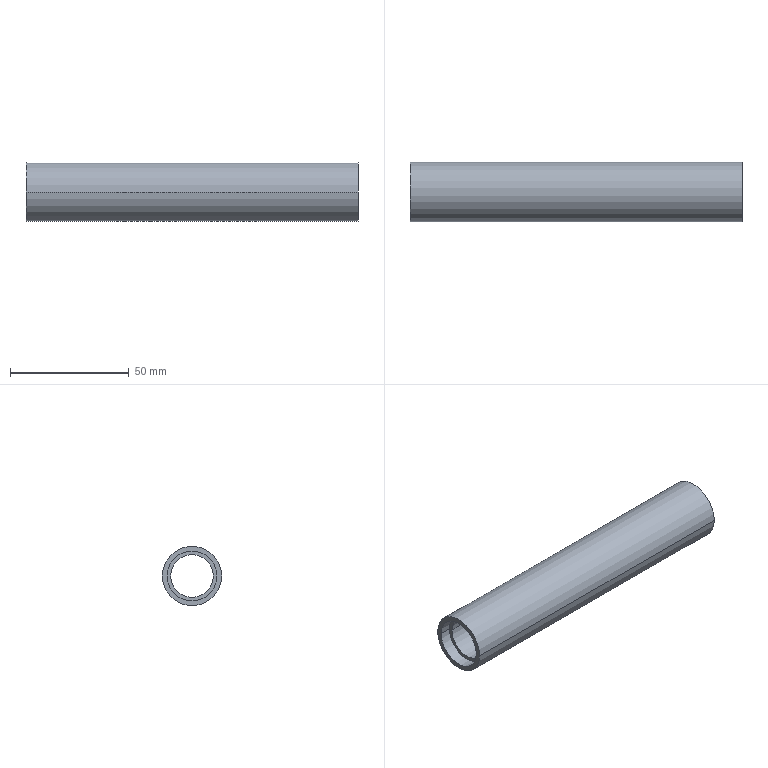Component | SolidWorks | IdlerAssembly4-1_Roller3-1 | 1 solid | 12 faces | box 140 x 25 x 25 mm | volume 32178 mm3 | cylinder 8 | plane 4 | commonest cylinder face diameters 21 x4 18 x2 25 x2
build123d program:
from build123d import *


with BuildPart() as part:
    # Sketch1 → Revolve1 (revolve)
    with BuildSketch(Plane.XY, mode=Mode.PRIVATE) as revolve1_sk:
        Polygon((0, 10.5), (5, 10.5), (5, 9), (135, 9), (135, 10.5), (140, 10.5), (140, 12.5), (0, 12.5), align=None)
    revolve(revolve1_sk.sketch.rotate(Axis((-1300.924, 0, 0), (1, 0, 0)), 90), axis=Axis((-1300.924, 0, 0), (1, 0, 0)))


solid = part.part

# Placed as in the assembly
solid = solid.moved(Location((-314.97, -95, 30), (0, 0, 0)))
STEP:
#1=CARTESIAN_POINT('',(-12.204,-3.327,1.181));
#2=VERTEX_POINT('',#1);
#3=CARTESIAN_POINT('',(-12.204,-4.154,1.181));
#4=VERTEX_POINT('',#3);
#5=CARTESIAN_POINT('',(-12.204,-3.74,1.181));
#6=DIRECTION('',(-1.,-0.,0.));
#7=DIRECTION('',(0.,-1.,0.));
#8=AXIS2_PLACEMENT_3D('',#5,#6,#7);
#9=CIRCLE('',#8,0.4134);
#10=EDGE_CURVE('',#2,#4,#9,.T.);
#11=ORIENTED_EDGE('',*,*,#10,.F.);
#12=CARTESIAN_POINT('',(-12.4,-3.327,1.181));
#13=VERTEX_POINT('',#12);
#14=CARTESIAN_POINT('',(-63.618,-3.327,1.181));
#15=DIRECTION('',(-1.,-0.,0.));
#16=VECTOR('',#15,39.37);
#17=LINE('',#14,#16);
#18=EDGE_CURVE('',#2,#13,#17,.T.);
#19=ORIENTED_EDGE('',*,*,#18,.T.);
#20=CARTESIAN_POINT('',(-12.4,-4.154,1.181));
#21=VERTEX_POINT('',#20);
#22=CARTESIAN_POINT('',(-12.4,-3.74,1.181));
#23=DIRECTION('',(-1.,-0.,0.));
#24=DIRECTION('',(0.,-1.,0.));
#25=AXIS2_PLACEMENT_3D('',#22,#23,#24);
#26=CIRCLE('',#25,0.4134);
#27=EDGE_CURVE('',#13,#21,#26,.T.);
#28=ORIENTED_EDGE('',*,*,#27,.T.);
#29=CARTESIAN_POINT('',(-63.618,-4.154,1.181));
#30=DIRECTION('',(-1.,-0.,0.));
#31=VECTOR('',#30,39.37);
#32=LINE('',#29,#31);
#33=EDGE_CURVE('',#4,#21,#32,.T.);
#34=ORIENTED_EDGE('',*,*,#33,.F.);
#35=EDGE_LOOP('',(#11,#19,#28,#34));
#36=FACE_OUTER_BOUND('',#35,.T.);
#37=CARTESIAN_POINT('',(-63.618,-3.74,1.181));
#38=DIRECTION('',(-1.,-0.,0.));
#39=DIRECTION('',(0.,-1.,0.));
#40=AXIS2_PLACEMENT_3D('',#37,#38,#39);
#41=CYLINDRICAL_SURFACE('',#40,0.4134);
#42=ADVANCED_FACE('',(#36),#41,.F.);
#43=CARTESIAN_POINT('',(-7.085,-3.386,1.181));
#44=VERTEX_POINT('',#43);
#45=CARTESIAN_POINT('',(-7.085,-4.094,1.181));
#46=VERTEX_POINT('',#45);
#47=CARTESIAN_POINT('',(-7.085,-3.74,1.181));
#48=DIRECTION('',(-1.,-0.,0.));
#49=DIRECTION('',(0.,-1.,0.));
#50=AXIS2_PLACEMENT_3D('',#47,#48,#49);
#51=CIRCLE('',#50,0.3543);
#52=EDGE_CURVE('',#44,#46,#51,.T.);
#53=ORIENTED_EDGE('',*,*,#52,.F.);
#54=CARTESIAN_POINT('',(-12.204,-3.386,1.181));
#55=VERTEX_POINT('',#54);
#56=CARTESIAN_POINT('',(-63.618,-3.386,1.181));
#57=DIRECTION('',(-1.,-0.,0.));
#58=VECTOR('',#57,39.37);
#59=LINE('',#56,#58);
#60=EDGE_CURVE('',#44,#55,#59,.T.);
#61=ORIENTED_EDGE('',*,*,#60,.T.);
#62=CARTESIAN_POINT('',(-12.204,-4.094,1.181));
#63=VERTEX_POINT('',#62);
#64=CARTESIAN_POINT('',(-12.204,-3.74,1.181));
#65=DIRECTION('',(-1.,-0.,0.));
#66=DIRECTION('',(0.,-1.,0.));
#67=AXIS2_PLACEMENT_3D('',#64,#65,#66);
#68=CIRCLE('',#67,0.3543);
#69=EDGE_CURVE('',#55,#63,#68,.T.);
#70=ORIENTED_EDGE('',*,*,#69,.T.);
#71=CARTESIAN_POINT('',(-63.618,-4.094,1.181));
#72=DIRECTION('',(-1.,-0.,0.));
#73=VECTOR('',#72,39.37);
#74=LINE('',#71,#73);
#75=EDGE_CURVE('',#46,#63,#74,.T.);
#76=ORIENTED_EDGE('',*,*,#75,.F.);
#77=EDGE_LOOP('',(#53,#61,#70,#76));
#78=FACE_OUTER_BOUND('',#77,.T.);
#79=CARTESIAN_POINT('',(-63.618,-3.74,1.181));
#80=DIRECTION('',(-1.,-0.,0.));
#81=DIRECTION('',(0.,-1.,0.));
#82=AXIS2_PLACEMENT_3D('',#79,#80,#81);
#83=CYLINDRICAL_SURFACE('',#82,0.3543);
#84=ADVANCED_FACE('',(#78),#83,.F.);
#85=CARTESIAN_POINT('',(-6.889,-3.327,1.181));
#86=VERTEX_POINT('',#85);
#87=CARTESIAN_POINT('',(-6.889,-4.154,1.181));
#88=VERTEX_POINT('',#87);
#89=CARTESIAN_POINT('',(-6.889,-3.74,1.181));
#90=DIRECTION('',(-1.,-0.,0.));
#91=DIRECTION('',(0.,-1.,0.));
#92=AXIS2_PLACEMENT_3D('',#89,#90,#91);
#93=CIRCLE('',#92,0.4134);
#94=EDGE_CURVE('',#86,#88,#93,.T.);
#95=ORIENTED_EDGE('',*,*,#94,.F.);
#96=CARTESIAN_POINT('',(-7.085,-3.327,1.181));
#97=VERTEX_POINT('',#96);
#98=CARTESIAN_POINT('',(-63.618,-3.327,1.181));
#99=DIRECTION('',(-1.,-0.,0.));
#100=VECTOR('',#99,39.37);
#101=LINE('',#98,#100);
#102=EDGE_CURVE('',#86,#97,#101,.T.);
#103=ORIENTED_EDGE('',*,*,#102,.T.);
#104=CARTESIAN_POINT('',(-7.085,-4.154,1.181));
#105=VERTEX_POINT('',#104);
#106=CARTESIAN_POINT('',(-7.085,-3.74,1.181));
#107=DIRECTION('',(-1.,-0.,0.));
#108=DIRECTION('',(0.,-1.,0.));
#109=AXIS2_PLACEMENT_3D('',#106,#107,#108);
#110=CIRCLE('',#109,0.4134);
#111=EDGE_CURVE('',#97,#105,#110,.T.);
#112=ORIENTED_EDGE('',*,*,#111,.T.);
#113=CARTESIAN_POINT('',(-63.618,-4.154,1.181));
#114=DIRECTION('',(-1.,-0.,0.));
#115=VECTOR('',#114,39.37);
#116=LINE('',#113,#115);
#117=EDGE_CURVE('',#88,#105,#116,.T.);
#118=ORIENTED_EDGE('',*,*,#117,.F.);
#119=EDGE_LOOP('',(#95,#103,#112,#118));
#120=FACE_OUTER_BOUND('',#119,.T.);
#121=CARTESIAN_POINT('',(-63.618,-3.74,1.181));
#122=DIRECTION('',(-1.,-0.,0.));
#123=DIRECTION('',(0.,-1.,0.));
#124=AXIS2_PLACEMENT_3D('',#121,#122,#123);
#125=CYLINDRICAL_SURFACE('',#124,0.4134);
#126=ADVANCED_FACE('',(#120),#125,.F.);
#127=CARTESIAN_POINT('',(-6.889,-4.232,1.181));
#128=VERTEX_POINT('',#127);
#129=CARTESIAN_POINT('',(-6.889,-3.248,1.181));
#130=VERTEX_POINT('',#129);
#131=CARTESIAN_POINT('',(-6.889,-3.74,1.181));
#132=DIRECTION('',(-1.,-0.,0.));
#133=DIRECTION('',(0.,-1.,0.));
#134=AXIS2_PLACEMENT_3D('',#131,#132,#133);
#135=CIRCLE('',#134,0.4921);
#136=EDGE_CURVE('',#128,#130,#135,.T.);
#137=ORIENTED_EDGE('',*,*,#136,.T.);
#138=CARTESIAN_POINT('',(-12.4,-3.248,1.181));
#139=VERTEX_POINT('',#138);
#140=CARTESIAN_POINT('',(-63.618,-3.248,1.181));
#141=DIRECTION('',(-1.,-0.,0.));
#142=VECTOR('',#141,39.37);
#143=LINE('',#140,#142);
#144=EDGE_CURVE('',#130,#139,#143,.T.);
#145=ORIENTED_EDGE('',*,*,#144,.T.);
#146=CARTESIAN_POINT('',(-12.4,-4.232,1.181));
#147=VERTEX_POINT('',#146);
#148=CARTESIAN_POINT('',(-12.4,-3.74,1.181));
#149=DIRECTION('',(-1.,-0.,0.));
#150=DIRECTION('',(0.,-1.,0.));
#151=AXIS2_PLACEMENT_3D('',#148,#149,#150);
#152=CIRCLE('',#151,0.4921);
#153=EDGE_CURVE('',#147,#139,#152,.T.);
#154=ORIENTED_EDGE('',*,*,#153,.F.);
#155=CARTESIAN_POINT('',(-63.618,-4.232,1.181));
#156=DIRECTION('',(-1.,-0.,0.));
#157=VECTOR('',#156,39.37);
#158=LINE('',#155,#157);
#159=EDGE_CURVE('',#128,#147,#158,.T.);
#160=ORIENTED_EDGE('',*,*,#159,.F.);
#161=EDGE_LOOP('',(#137,#145,#154,#160));
#162=FACE_OUTER_BOUND('',#161,.T.);
#163=CARTESIAN_POINT('',(-63.618,-3.74,1.181));
#164=DIRECTION('',(-1.,-0.,0.));
#165=DIRECTION('',(0.,-1.,0.));
#166=AXIS2_PLACEMENT_3D('',#163,#164,#165);
#167=CYLINDRICAL_SURFACE('',#166,0.4921);
#168=ADVANCED_FACE('',(#162),#167,.T.);
#169=CARTESIAN_POINT('',(-12.4,-3.74,1.181));
#170=DIRECTION('',(-1.,-0.,0.));
#171=DIRECTION('',(0.,-1.,0.));
#172=AXIS2_PLACEMENT_3D('',#169,#170,#171);
#173=CIRCLE('',#172,0.4134);
#174=EDGE_CURVE('',#21,#13,#173,.T.);
#175=ORIENTED_EDGE('',*,*,#174,.F.);
#176=ORIENTED_EDGE('',*,*,#27,.F.);
#177=EDGE_LOOP('',(#175,#176));
#178=FACE_BOUND('',#177,.T.);
#179=ORIENTED_EDGE('',*,*,#153,.T.);
#180=CARTESIAN_POINT('',(-12.4,-3.74,1.181));
#181=DIRECTION('',(-1.,-0.,0.));
#182=DIRECTION('',(0.,-1.,0.));
#183=AXIS2_PLACEMENT_3D('',#180,#181,#182);
#184=CIRCLE('',#183,0.4921);
#185=EDGE_CURVE('',#139,#147,#184,.T.);
#186=ORIENTED_EDGE('',*,*,#185,.T.);
#187=EDGE_LOOP('',(#179,#186));
#188=FACE_OUTER_BOUND('',#187,.T.);
#189=CARTESIAN_POINT('',(-12.4,-3.74,1.594));
#190=DIRECTION('',(1.,0.,-0.));
#191=DIRECTION('',(-0.,1.,0.));
#192=AXIS2_PLACEMENT_3D('',#189,#190,#191);
#193=PLANE('',#192);
#194=ADVANCED_FACE('',(#178,#188),#193,.F.);
#195=ORIENTED_EDGE('',*,*,#144,.F.);
#196=CARTESIAN_POINT('',(-6.889,-3.74,1.181));
#197=DIRECTION('',(-1.,-0.,0.));
#198=DIRECTION('',(0.,-1.,0.));
#199=AXIS2_PLACEMENT_3D('',#196,#197,#198);
#200=CIRCLE('',#199,0.4921);
#201=EDGE_CURVE('',#130,#128,#200,.T.);
#202=ORIENTED_EDGE('',*,*,#201,.T.);
#203=ORIENTED_EDGE('',*,*,#159,.T.);
#204=ORIENTED_EDGE('',*,*,#185,.F.);
#205=EDGE_LOOP('',(#195,#202,#203,#204));
#206=FACE_OUTER_BOUND('',#205,.T.);
#207=CARTESIAN_POINT('',(-63.618,-3.74,1.181));
#208=DIRECTION('',(-1.,-0.,0.));
#209=DIRECTION('',(0.,-1.,0.));
#210=AXIS2_PLACEMENT_3D('',#207,#208,#209);
#211=CYLINDRICAL_SURFACE('',#210,0.4921);
#212=ADVANCED_FACE('',(#206),#211,.T.);
#213=ORIENTED_EDGE('',*,*,#136,.F.);
#214=ORIENTED_EDGE('',*,*,#201,.F.);
#215=EDGE_LOOP('',(#213,#214));
#216=FACE_OUTER_BOUND('',#215,.T.);
#217=CARTESIAN_POINT('',(-6.889,-3.74,1.181));
#218=DIRECTION('',(-1.,-0.,0.));
#219=DIRECTION('',(0.,-1.,0.));
#220=AXIS2_PLACEMENT_3D('',#217,#218,#219);
#221=CIRCLE('',#220,0.4134);
#222=EDGE_CURVE('',#88,#86,#221,.T.);
#223=ORIENTED_EDGE('',*,*,#222,.T.);
#224=ORIENTED_EDGE('',*,*,#94,.T.);
#225=EDGE_LOOP('',(#223,#224));
#226=FACE_BOUND('',#225,.T.);
#227=CARTESIAN_POINT('',(-6.889,-3.74,1.673));
#228=DIRECTION('',(-1.,-0.,0.));
#229=DIRECTION('',(0.,-1.,0.));
#230=AXIS2_PLACEMENT_3D('',#227,#228,#229);
#231=PLANE('',#230);
#232=ADVANCED_FACE('',(#216,#226),#231,.F.);
#233=ORIENTED_EDGE('',*,*,#102,.F.);
#234=ORIENTED_EDGE('',*,*,#222,.F.);
#235=ORIENTED_EDGE('',*,*,#117,.T.);
#236=CARTESIAN_POINT('',(-7.085,-3.74,1.181));
#237=DIRECTION('',(-1.,-0.,0.));
#238=DIRECTION('',(0.,-1.,0.));
#239=AXIS2_PLACEMENT_3D('',#236,#237,#238);
#240=CIRCLE('',#239,0.4134);
#241=EDGE_CURVE('',#105,#97,#240,.T.);
#242=ORIENTED_EDGE('',*,*,#241,.T.);
#243=EDGE_LOOP('',(#233,#234,#235,#242));
#244=FACE_OUTER_BOUND('',#243,.T.);
#245=CARTESIAN_POINT('',(-63.618,-3.74,1.181));
#246=DIRECTION('',(-1.,-0.,0.));
#247=DIRECTION('',(0.,-1.,0.));
#248=AXIS2_PLACEMENT_3D('',#245,#246,#247);
#249=CYLINDRICAL_SURFACE('',#248,0.4134);
#250=ADVANCED_FACE('',(#244),#249,.F.);
#251=ORIENTED_EDGE('',*,*,#241,.F.);
#252=ORIENTED_EDGE('',*,*,#111,.F.);
#253=EDGE_LOOP('',(#251,#252));
#254=FACE_OUTER_BOUND('',#253,.T.);
#255=CARTESIAN_POINT('',(-7.085,-3.74,1.181));
#256=DIRECTION('',(-1.,-0.,0.));
#257=DIRECTION('',(0.,-1.,0.));
#258=AXIS2_PLACEMENT_3D('',#255,#256,#257);
#259=CIRCLE('',#258,0.3543);
#260=EDGE_CURVE('',#46,#44,#259,.T.);
#261=ORIENTED_EDGE('',*,*,#260,.T.);
#262=ORIENTED_EDGE('',*,*,#52,.T.);
#263=EDGE_LOOP('',(#261,#262));
#264=FACE_BOUND('',#263,.T.);
#265=CARTESIAN_POINT('',(-7.085,-3.74,1.535));
#266=DIRECTION('',(-1.,-0.,0.));
#267=DIRECTION('',(0.,-1.,0.));
#268=AXIS2_PLACEMENT_3D('',#265,#266,#267);
#269=PLANE('',#268);
#270=ADVANCED_FACE('',(#254,#264),#269,.F.);
#271=ORIENTED_EDGE('',*,*,#60,.F.);
#272=ORIENTED_EDGE('',*,*,#260,.F.);
#273=ORIENTED_EDGE('',*,*,#75,.T.);
#274=CARTESIAN_POINT('',(-12.204,-3.74,1.181));
#275=DIRECTION('',(-1.,-0.,0.));
#276=DIRECTION('',(0.,-1.,0.));
#277=AXIS2_PLACEMENT_3D('',#274,#275,#276);
#278=CIRCLE('',#277,0.3543);
#279=EDGE_CURVE('',#63,#55,#278,.T.);
#280=ORIENTED_EDGE('',*,*,#279,.T.);
#281=EDGE_LOOP('',(#271,#272,#273,#280));
#282=FACE_OUTER_BOUND('',#281,.T.);
#283=CARTESIAN_POINT('',(-63.618,-3.74,1.181));
#284=DIRECTION('',(-1.,-0.,0.));
#285=DIRECTION('',(0.,-1.,0.));
#286=AXIS2_PLACEMENT_3D('',#283,#284,#285);
#287=CYLINDRICAL_SURFACE('',#286,0.3543);
#288=ADVANCED_FACE('',(#282),#287,.F.);
#289=ORIENTED_EDGE('',*,*,#279,.F.);
#290=ORIENTED_EDGE('',*,*,#69,.F.);
#291=EDGE_LOOP('',(#289,#290));
#292=FACE_BOUND('',#291,.T.);
#293=CARTESIAN_POINT('',(-12.204,-3.74,1.181));
#294=DIRECTION('',(-1.,-0.,0.));
#295=DIRECTION('',(0.,-1.,0.));
#296=AXIS2_PLACEMENT_3D('',#293,#294,#295);
#297=CIRCLE('',#296,0.4134);
#298=EDGE_CURVE('',#4,#2,#297,.T.);
#299=ORIENTED_EDGE('',*,*,#298,.T.);
#300=ORIENTED_EDGE('',*,*,#10,.T.);
#301=EDGE_LOOP('',(#299,#300));
#302=FACE_OUTER_BOUND('',#301,.T.);
#303=CARTESIAN_POINT('',(-12.204,-3.74,1.594));
#304=DIRECTION('',(1.,0.,-0.));
#305=DIRECTION('',(-0.,1.,0.));
#306=AXIS2_PLACEMENT_3D('',#303,#304,#305);
#307=PLANE('',#306);
#308=ADVANCED_FACE('',(#292,#302),#307,.F.);
#309=ORIENTED_EDGE('',*,*,#18,.F.);
#310=ORIENTED_EDGE('',*,*,#298,.F.);
#311=ORIENTED_EDGE('',*,*,#33,.T.);
#312=ORIENTED_EDGE('',*,*,#174,.T.);
#313=EDGE_LOOP('',(#309,#310,#311,#312));
#314=FACE_OUTER_BOUND('',#313,.T.);
#315=CARTESIAN_POINT('',(-63.618,-3.74,1.181));
#316=DIRECTION('',(-1.,-0.,0.));
#317=DIRECTION('',(0.,-1.,0.));
#318=AXIS2_PLACEMENT_3D('',#315,#316,#317);
#319=CYLINDRICAL_SURFACE('',#318,0.4134);
#320=ADVANCED_FACE('',(#314),#319,.F.);
#321=CLOSED_SHELL('',(#42,#84,#126,#168,#194,#212,#232,#250,#270,#288,#308,#320));
#322=MANIFOLD_SOLID_BREP('',#321);
#323=CARTESIAN_POINT('',(0.,0.,0.));
#324=DIRECTION('',(0.,0.,1.));
#325=DIRECTION('',(1.,0.,0.));
#326=AXIS2_PLACEMENT_3D('',#323,#324,#325);
#327=(LENGTH_UNIT()NAMED_UNIT(*)SI_UNIT($,.METRE.));
#328=LENGTH_MEASURE_WITH_UNIT(LENGTH_MEASURE(0.0254),#327);
#329=DIMENSIONAL_EXPONENTS(1.,0.,0.,0.,0.,0.,0.);
#330=(CONVERSION_BASED_UNIT('',#328)LENGTH_UNIT()NAMED_UNIT(#329));
#331=UNCERTAINTY_MEASURE_WITH_UNIT(LENGTH_MEASURE(0.00001),#330,'','');
#332=(NAMED_UNIT(*)PLANE_ANGLE_UNIT()SI_UNIT($,.RADIAN.));
#333=(NAMED_UNIT(*)SI_UNIT($,.STERADIAN.)SOLID_ANGLE_UNIT());
#334=(GEOMETRIC_REPRESENTATION_CONTEXT(3)GLOBAL_UNCERTAINTY_ASSIGNED_CONTEXT((#331))GLOBAL_UNIT_ASSIGNED_CONTEXT((#330,#332,#333))REPRESENTATION_CONTEXT('',''));
#335=ADVANCED_BREP_SHAPE_REPRESENTATION('',(#322,#326),#334);
#336=COLOUR_RGB('',0.7922,0.8196,0.9333);
#337=FILL_AREA_STYLE_COLOUR('',#336);
#338=FILL_AREA_STYLE('',(#337));
#339=SURFACE_STYLE_FILL_AREA(#338);
#340=SURFACE_SIDE_STYLE('',(#339));
#341=SURFACE_STYLE_USAGE(.BOTH.,#340);
#342=PRESENTATION_STYLE_ASSIGNMENT((#341));
#343=STYLED_ITEM('',(#342),#322);
#344=PRESENTATION_LAYER_ASSIGNMENT('','',(#343));
#345=(LENGTH_UNIT()NAMED_UNIT(*)SI_UNIT($,.METRE.));
#346=LENGTH_MEASURE_WITH_UNIT(LENGTH_MEASURE(0.0254),#345);
#347=DIMENSIONAL_EXPONENTS(1.,0.,0.,0.,0.,0.,0.);
#348=(CONVERSION_BASED_UNIT('',#346)LENGTH_UNIT()NAMED_UNIT(#347));
#349=UNCERTAINTY_MEASURE_WITH_UNIT(LENGTH_MEASURE(0.00001),#348,'','');
#350=(NAMED_UNIT(*)PLANE_ANGLE_UNIT()SI_UNIT($,.RADIAN.));
#351=(NAMED_UNIT(*)SI_UNIT($,.STERADIAN.)SOLID_ANGLE_UNIT());
#352=(GEOMETRIC_REPRESENTATION_CONTEXT(3)GLOBAL_UNCERTAINTY_ASSIGNED_CONTEXT((#349))GLOBAL_UNIT_ASSIGNED_CONTEXT((#348,#350,#351))REPRESENTATION_CONTEXT('',''));
#353=MECHANICAL_DESIGN_GEOMETRIC_PRESENTATION_REPRESENTATION('',(#343),#352);